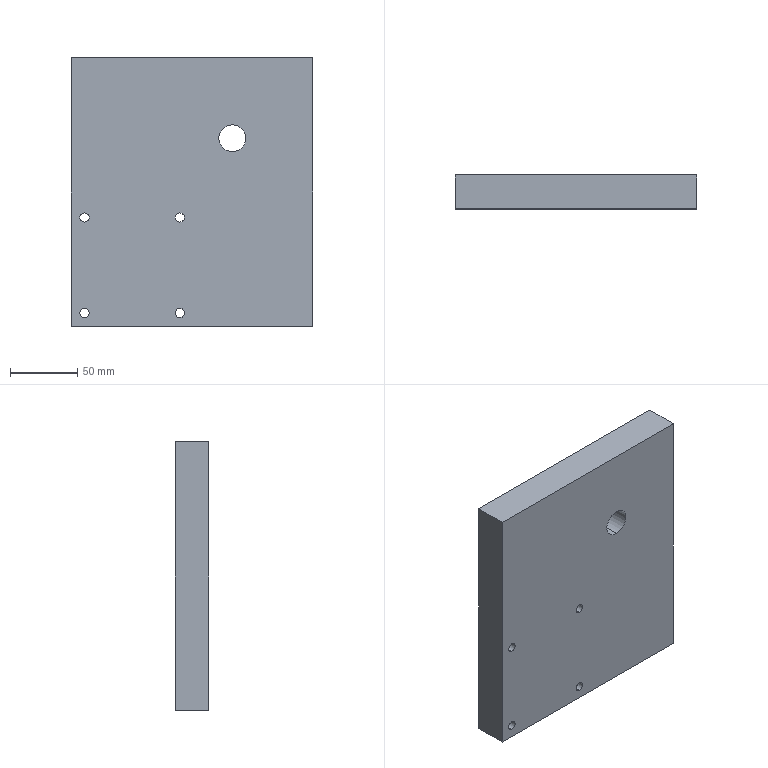Component | SolidWorks | 30-01A-1_Wheel-322-1_WheelFixingPlate-322-1 | 1 solid | 16 faces | box 180 x 25 x 200 mm | volume 888514 mm3 | cylinder 10 | plane 6 | commonest cylinder face diameters 6.8 x8 20 x2
build123d program:
from build123d import *

# Parameters (mm, degrees)
SKETCH1_W              = 200
SKETCH1_H              = 180
EXTRUDE1_DEPTH         = 12.5
M20X2_5_TAPPED_HOLE1_D = 20
M8X1_25_TAPPED_HOLE1_D = 6.8


with BuildPart() as part:
    # Sketch1 → Extrude1 (new, symmetric)
    with BuildSketch(Plane.XY):
        Rectangle(SKETCH1_W, SKETCH1_H)
    extrude(amount=EXTRUDE1_DEPTH, both=True)

    # M20x2.5 Tapped Hole1 (through all)
    with Locations(Plane.XY.offset(12.5)):
        with Locations((-40, -30)):
            Hole(M20X2_5_TAPPED_HOLE1_D / 2)

    # M8x1.25 Tapped Hole1 (through all)
    with Locations(Plane.XY.offset(12.5)):
        with Locations((19, 9), (90, 9), (90, 80), (19, 80)):
            Hole(M8X1_25_TAPPED_HOLE1_D / 2)


solid = part.part

# Placed as in the assembly
solid = solid.moved(Location((202.57, -550.345, -60), (-90, 0, 90)))
STEP:
#1=CARTESIAN_POINT('',(7.621,-22.159,-2.976));
#2=VERTEX_POINT('',#1);
#3=CARTESIAN_POINT('',(7.621,-22.159,-3.244));
#4=VERTEX_POINT('',#3);
#5=CARTESIAN_POINT('',(7.621,-22.159,-3.11));
#6=DIRECTION('',(0.,1.,-0.));
#7=DIRECTION('',(0.,0.,-1.));
#8=AXIS2_PLACEMENT_3D('',#5,#6,#7);
#9=CIRCLE('',#8,0.1339);
#10=EDGE_CURVE('',#2,#4,#9,.T.);
#11=ORIENTED_EDGE('',*,*,#10,.F.);
#12=CARTESIAN_POINT('',(7.621,-21.175,-2.976));
#13=VERTEX_POINT('',#12);
#14=CARTESIAN_POINT('',(7.621,-21.175,-2.976));
#15=DIRECTION('',(0.,1.,-0.));
#16=VECTOR('',#15,39.37);
#17=LINE('',#14,#16);
#18=EDGE_CURVE('',#2,#13,#17,.T.);
#19=ORIENTED_EDGE('',*,*,#18,.T.);
#20=CARTESIAN_POINT('',(7.621,-21.175,-3.244));
#21=VERTEX_POINT('',#20);
#22=CARTESIAN_POINT('',(7.621,-21.175,-3.11));
#23=DIRECTION('',(0.,1.,-0.));
#24=DIRECTION('',(0.,0.,-1.));
#25=AXIS2_PLACEMENT_3D('',#22,#23,#24);
#26=CIRCLE('',#25,0.1339);
#27=EDGE_CURVE('',#13,#21,#26,.T.);
#28=ORIENTED_EDGE('',*,*,#27,.T.);
#29=CARTESIAN_POINT('',(7.621,-21.175,-3.244));
#30=DIRECTION('',(0.,1.,-0.));
#31=VECTOR('',#30,39.37);
#32=LINE('',#29,#31);
#33=EDGE_CURVE('',#4,#21,#32,.T.);
#34=ORIENTED_EDGE('',*,*,#33,.F.);
#35=EDGE_LOOP('',(#11,#19,#28,#34));
#36=FACE_OUTER_BOUND('',#35,.T.);
#37=CARTESIAN_POINT('',(7.621,-21.175,-3.11));
#38=DIRECTION('',(0.,1.,-0.));
#39=DIRECTION('',(0.,0.,-1.));
#40=AXIS2_PLACEMENT_3D('',#37,#38,#39);
#41=CYLINDRICAL_SURFACE('',#40,0.1339);
#42=ADVANCED_FACE('',(#36),#41,.F.);
#43=CARTESIAN_POINT('',(7.621,-22.159,-5.772));
#44=VERTEX_POINT('',#43);
#45=CARTESIAN_POINT('',(7.621,-22.159,-6.039));
#46=VERTEX_POINT('',#45);
#47=CARTESIAN_POINT('',(7.621,-22.159,-5.906));
#48=DIRECTION('',(0.,1.,-0.));
#49=DIRECTION('',(0.,0.,-1.));
#50=AXIS2_PLACEMENT_3D('',#47,#48,#49);
#51=CIRCLE('',#50,0.1339);
#52=EDGE_CURVE('',#44,#46,#51,.T.);
#53=ORIENTED_EDGE('',*,*,#52,.F.);
#54=CARTESIAN_POINT('',(7.621,-21.175,-5.772));
#55=VERTEX_POINT('',#54);
#56=CARTESIAN_POINT('',(7.621,-21.175,-5.772));
#57=DIRECTION('',(0.,1.,-0.));
#58=VECTOR('',#57,39.37);
#59=LINE('',#56,#58);
#60=EDGE_CURVE('',#44,#55,#59,.T.);
#61=ORIENTED_EDGE('',*,*,#60,.T.);
#62=CARTESIAN_POINT('',(7.621,-21.175,-6.039));
#63=VERTEX_POINT('',#62);
#64=CARTESIAN_POINT('',(7.621,-21.175,-5.906));
#65=DIRECTION('',(0.,1.,-0.));
#66=DIRECTION('',(0.,0.,-1.));
#67=AXIS2_PLACEMENT_3D('',#64,#65,#66);
#68=CIRCLE('',#67,0.1339);
#69=EDGE_CURVE('',#55,#63,#68,.T.);
#70=ORIENTED_EDGE('',*,*,#69,.T.);
#71=CARTESIAN_POINT('',(7.621,-21.175,-6.039));
#72=DIRECTION('',(0.,1.,-0.));
#73=VECTOR('',#72,39.37);
#74=LINE('',#71,#73);
#75=EDGE_CURVE('',#46,#63,#74,.T.);
#76=ORIENTED_EDGE('',*,*,#75,.F.);
#77=EDGE_LOOP('',(#53,#61,#70,#76));
#78=FACE_OUTER_BOUND('',#77,.T.);
#79=CARTESIAN_POINT('',(7.621,-21.175,-5.906));
#80=DIRECTION('',(0.,1.,-0.));
#81=DIRECTION('',(0.,0.,-1.));
#82=AXIS2_PLACEMENT_3D('',#79,#80,#81);
#83=CYLINDRICAL_SURFACE('',#82,0.1339);
#84=ADVANCED_FACE('',(#78),#83,.F.);
#85=CARTESIAN_POINT('',(4.826,-22.159,-5.772));
#86=VERTEX_POINT('',#85);
#87=CARTESIAN_POINT('',(4.826,-22.159,-6.039));
#88=VERTEX_POINT('',#87);
#89=CARTESIAN_POINT('',(4.826,-22.159,-5.906));
#90=DIRECTION('',(0.,1.,-0.));
#91=DIRECTION('',(0.,0.,-1.));
#92=AXIS2_PLACEMENT_3D('',#89,#90,#91);
#93=CIRCLE('',#92,0.1339);
#94=EDGE_CURVE('',#86,#88,#93,.T.);
#95=ORIENTED_EDGE('',*,*,#94,.F.);
#96=CARTESIAN_POINT('',(4.826,-21.175,-5.772));
#97=VERTEX_POINT('',#96);
#98=CARTESIAN_POINT('',(4.826,-21.175,-5.772));
#99=DIRECTION('',(0.,1.,-0.));
#100=VECTOR('',#99,39.37);
#101=LINE('',#98,#100);
#102=EDGE_CURVE('',#86,#97,#101,.T.);
#103=ORIENTED_EDGE('',*,*,#102,.T.);
#104=CARTESIAN_POINT('',(4.826,-21.175,-6.039));
#105=VERTEX_POINT('',#104);
#106=CARTESIAN_POINT('',(4.826,-21.175,-5.906));
#107=DIRECTION('',(0.,1.,-0.));
#108=DIRECTION('',(0.,0.,-1.));
#109=AXIS2_PLACEMENT_3D('',#106,#107,#108);
#110=CIRCLE('',#109,0.1339);
#111=EDGE_CURVE('',#97,#105,#110,.T.);
#112=ORIENTED_EDGE('',*,*,#111,.T.);
#113=CARTESIAN_POINT('',(4.826,-21.175,-6.039));
#114=DIRECTION('',(0.,1.,-0.));
#115=VECTOR('',#114,39.37);
#116=LINE('',#113,#115);
#117=EDGE_CURVE('',#88,#105,#116,.T.);
#118=ORIENTED_EDGE('',*,*,#117,.F.);
#119=EDGE_LOOP('',(#95,#103,#112,#118));
#120=FACE_OUTER_BOUND('',#119,.T.);
#121=CARTESIAN_POINT('',(4.826,-21.175,-5.906));
#122=DIRECTION('',(0.,1.,-0.));
#123=DIRECTION('',(0.,0.,-1.));
#124=AXIS2_PLACEMENT_3D('',#121,#122,#123);
#125=CYLINDRICAL_SURFACE('',#124,0.1339);
#126=ADVANCED_FACE('',(#120),#125,.F.);
#127=CARTESIAN_POINT('',(4.826,-22.159,-2.976));
#128=VERTEX_POINT('',#127);
#129=CARTESIAN_POINT('',(4.826,-22.159,-3.244));
#130=VERTEX_POINT('',#129);
#131=CARTESIAN_POINT('',(4.826,-22.159,-3.11));
#132=DIRECTION('',(0.,1.,-0.));
#133=DIRECTION('',(0.,0.,-1.));
#134=AXIS2_PLACEMENT_3D('',#131,#132,#133);
#135=CIRCLE('',#134,0.1339);
#136=EDGE_CURVE('',#128,#130,#135,.T.);
#137=ORIENTED_EDGE('',*,*,#136,.F.);
#138=CARTESIAN_POINT('',(4.826,-21.175,-2.976));
#139=VERTEX_POINT('',#138);
#140=CARTESIAN_POINT('',(4.826,-21.175,-2.976));
#141=DIRECTION('',(0.,1.,-0.));
#142=VECTOR('',#141,39.37);
#143=LINE('',#140,#142);
#144=EDGE_CURVE('',#128,#139,#143,.T.);
#145=ORIENTED_EDGE('',*,*,#144,.T.);
#146=CARTESIAN_POINT('',(4.826,-21.175,-3.244));
#147=VERTEX_POINT('',#146);
#148=CARTESIAN_POINT('',(4.826,-21.175,-3.11));
#149=DIRECTION('',(0.,1.,-0.));
#150=DIRECTION('',(0.,0.,-1.));
#151=AXIS2_PLACEMENT_3D('',#148,#149,#150);
#152=CIRCLE('',#151,0.1339);
#153=EDGE_CURVE('',#139,#147,#152,.T.);
#154=ORIENTED_EDGE('',*,*,#153,.T.);
#155=CARTESIAN_POINT('',(4.826,-21.175,-3.244));
#156=DIRECTION('',(0.,1.,-0.));
#157=VECTOR('',#156,39.37);
#158=LINE('',#155,#157);
#159=EDGE_CURVE('',#130,#147,#158,.T.);
#160=ORIENTED_EDGE('',*,*,#159,.F.);
#161=EDGE_LOOP('',(#137,#145,#154,#160));
#162=FACE_OUTER_BOUND('',#161,.T.);
#163=CARTESIAN_POINT('',(4.826,-21.175,-3.11));
#164=DIRECTION('',(0.,1.,-0.));
#165=DIRECTION('',(0.,0.,-1.));
#166=AXIS2_PLACEMENT_3D('',#163,#164,#165);
#167=CYLINDRICAL_SURFACE('',#166,0.1339);
#168=ADVANCED_FACE('',(#162),#167,.F.);
#169=CARTESIAN_POINT('',(9.156,-22.159,-0.3937));
#170=VERTEX_POINT('',#169);
#171=CARTESIAN_POINT('',(9.156,-22.159,-1.181));
#172=VERTEX_POINT('',#171);
#173=CARTESIAN_POINT('',(9.156,-22.159,-0.7874));
#174=DIRECTION('',(0.,1.,-0.));
#175=DIRECTION('',(0.,0.,-1.));
#176=AXIS2_PLACEMENT_3D('',#173,#174,#175);
#177=CIRCLE('',#176,0.3937);
#178=EDGE_CURVE('',#170,#172,#177,.T.);
#179=ORIENTED_EDGE('',*,*,#178,.F.);
#180=CARTESIAN_POINT('',(9.156,-21.175,-0.3937));
#181=VERTEX_POINT('',#180);
#182=CARTESIAN_POINT('',(9.156,-21.175,-0.3937));
#183=DIRECTION('',(0.,1.,-0.));
#184=VECTOR('',#183,39.37);
#185=LINE('',#182,#184);
#186=EDGE_CURVE('',#170,#181,#185,.T.);
#187=ORIENTED_EDGE('',*,*,#186,.T.);
#188=CARTESIAN_POINT('',(9.156,-21.175,-1.181));
#189=VERTEX_POINT('',#188);
#190=CARTESIAN_POINT('',(9.156,-21.175,-0.7874));
#191=DIRECTION('',(0.,1.,-0.));
#192=DIRECTION('',(0.,0.,-1.));
#193=AXIS2_PLACEMENT_3D('',#190,#191,#192);
#194=CIRCLE('',#193,0.3937);
#195=EDGE_CURVE('',#181,#189,#194,.T.);
#196=ORIENTED_EDGE('',*,*,#195,.T.);
#197=CARTESIAN_POINT('',(9.156,-21.175,-1.181));
#198=DIRECTION('',(0.,1.,-0.));
#199=VECTOR('',#198,39.37);
#200=LINE('',#197,#199);
#201=EDGE_CURVE('',#172,#189,#200,.T.);
#202=ORIENTED_EDGE('',*,*,#201,.F.);
#203=EDGE_LOOP('',(#179,#187,#196,#202));
#204=FACE_OUTER_BOUND('',#203,.T.);
#205=CARTESIAN_POINT('',(9.156,-21.175,-0.7874));
#206=DIRECTION('',(0.,1.,-0.));
#207=DIRECTION('',(0.,0.,-1.));
#208=AXIS2_PLACEMENT_3D('',#205,#206,#207);
#209=CYLINDRICAL_SURFACE('',#208,0.3937);
#210=ADVANCED_FACE('',(#204),#209,.F.);
#211=CARTESIAN_POINT('',(4.432,-22.159,1.575));
#212=VERTEX_POINT('',#211);
#213=CARTESIAN_POINT('',(11.519,-22.159,1.575));
#214=VERTEX_POINT('',#213);
#215=CARTESIAN_POINT('',(4.432,-22.159,1.575));
#216=DIRECTION('',(1.,-0.,-0.));
#217=VECTOR('',#216,39.37);
#218=LINE('',#215,#217);
#219=EDGE_CURVE('',#212,#214,#218,.T.);
#220=ORIENTED_EDGE('',*,*,#219,.T.);
#221=CARTESIAN_POINT('',(11.519,-21.175,1.575));
#222=VERTEX_POINT('',#221);
#223=CARTESIAN_POINT('',(11.519,-21.175,1.575));
#224=DIRECTION('',(-0.,-1.,0.));
#225=VECTOR('',#224,39.37);
#226=LINE('',#223,#225);
#227=EDGE_CURVE('',#222,#214,#226,.T.);
#228=ORIENTED_EDGE('',*,*,#227,.F.);
#229=CARTESIAN_POINT('',(4.432,-21.175,1.575));
#230=VERTEX_POINT('',#229);
#231=CARTESIAN_POINT('',(4.432,-21.175,1.575));
#232=DIRECTION('',(1.,-0.,-0.));
#233=VECTOR('',#232,39.37);
#234=LINE('',#231,#233);
#235=EDGE_CURVE('',#230,#222,#234,.T.);
#236=ORIENTED_EDGE('',*,*,#235,.F.);
#237=CARTESIAN_POINT('',(4.432,-21.175,1.575));
#238=DIRECTION('',(-0.,-1.,0.));
#239=VECTOR('',#238,39.37);
#240=LINE('',#237,#239);
#241=EDGE_CURVE('',#230,#212,#240,.T.);
#242=ORIENTED_EDGE('',*,*,#241,.T.);
#243=EDGE_LOOP('',(#220,#228,#236,#242));
#244=FACE_OUTER_BOUND('',#243,.T.);
#245=CARTESIAN_POINT('',(4.432,-21.175,1.575));
#246=DIRECTION('',(-0.,-0.,-1.));
#247=DIRECTION('',(-0.,-1.,0.));
#248=AXIS2_PLACEMENT_3D('',#245,#246,#247);
#249=PLANE('',#248);
#250=ADVANCED_FACE('',(#244),#249,.F.);
#251=CARTESIAN_POINT('',(11.519,-22.159,-6.299));
#252=VERTEX_POINT('',#251);
#253=CARTESIAN_POINT('',(11.519,-22.159,1.575));
#254=DIRECTION('',(-0.,-0.,-1.));
#255=VECTOR('',#254,39.37);
#256=LINE('',#253,#255);
#257=EDGE_CURVE('',#214,#252,#256,.T.);
#258=ORIENTED_EDGE('',*,*,#257,.T.);
#259=CARTESIAN_POINT('',(11.519,-21.175,-6.299));
#260=VERTEX_POINT('',#259);
#261=CARTESIAN_POINT('',(11.519,-21.175,-6.299));
#262=DIRECTION('',(-0.,-1.,0.));
#263=VECTOR('',#262,39.37);
#264=LINE('',#261,#263);
#265=EDGE_CURVE('',#260,#252,#264,.T.);
#266=ORIENTED_EDGE('',*,*,#265,.F.);
#267=CARTESIAN_POINT('',(11.519,-21.175,1.575));
#268=DIRECTION('',(-0.,-0.,-1.));
#269=VECTOR('',#268,39.37);
#270=LINE('',#267,#269);
#271=EDGE_CURVE('',#222,#260,#270,.T.);
#272=ORIENTED_EDGE('',*,*,#271,.F.);
#273=ORIENTED_EDGE('',*,*,#227,.T.);
#274=EDGE_LOOP('',(#258,#266,#272,#273));
#275=FACE_OUTER_BOUND('',#274,.T.);
#276=CARTESIAN_POINT('',(11.519,-21.175,1.575));
#277=DIRECTION('',(-1.,0.,0.));
#278=DIRECTION('',(0.,1.,-0.));
#279=AXIS2_PLACEMENT_3D('',#276,#277,#278);
#280=PLANE('',#279);
#281=ADVANCED_FACE('',(#275),#280,.F.);
#282=CARTESIAN_POINT('',(4.432,-22.159,-6.299));
#283=VERTEX_POINT('',#282);
#284=CARTESIAN_POINT('',(4.432,-22.159,-6.299));
#285=DIRECTION('',(-1.,0.,0.));
#286=VECTOR('',#285,39.37);
#287=LINE('',#284,#286);
#288=EDGE_CURVE('',#252,#283,#287,.T.);
#289=ORIENTED_EDGE('',*,*,#288,.T.);
#290=CARTESIAN_POINT('',(4.432,-21.175,-6.299));
#291=VERTEX_POINT('',#290);
#292=CARTESIAN_POINT('',(4.432,-21.175,-6.299));
#293=DIRECTION('',(-0.,-1.,0.));
#294=VECTOR('',#293,39.37);
#295=LINE('',#292,#294);
#296=EDGE_CURVE('',#291,#283,#295,.T.);
#297=ORIENTED_EDGE('',*,*,#296,.F.);
#298=CARTESIAN_POINT('',(4.432,-21.175,-6.299));
#299=DIRECTION('',(-1.,0.,0.));
#300=VECTOR('',#299,39.37);
#301=LINE('',#298,#300);
#302=EDGE_CURVE('',#260,#291,#301,.T.);
#303=ORIENTED_EDGE('',*,*,#302,.F.);
#304=ORIENTED_EDGE('',*,*,#265,.T.);
#305=EDGE_LOOP('',(#289,#297,#303,#304));
#306=FACE_OUTER_BOUND('',#305,.T.);
#307=CARTESIAN_POINT('',(4.432,-21.175,-6.299));
#308=DIRECTION('',(0.,0.,1.));
#309=DIRECTION('',(0.,1.,-0.));
#310=AXIS2_PLACEMENT_3D('',#307,#308,#309);
#311=PLANE('',#310);
#312=ADVANCED_FACE('',(#306),#311,.F.);
#313=CARTESIAN_POINT('',(4.432,-22.159,1.575));
#314=DIRECTION('',(0.,0.,1.));
#315=VECTOR('',#314,39.37);
#316=LINE('',#313,#315);
#317=EDGE_CURVE('',#283,#212,#316,.T.);
#318=ORIENTED_EDGE('',*,*,#317,.T.);
#319=ORIENTED_EDGE('',*,*,#241,.F.);
#320=CARTESIAN_POINT('',(4.432,-21.175,1.575));
#321=DIRECTION('',(0.,0.,1.));
#322=VECTOR('',#321,39.37);
#323=LINE('',#320,#322);
#324=EDGE_CURVE('',#291,#230,#323,.T.);
#325=ORIENTED_EDGE('',*,*,#324,.F.);
#326=ORIENTED_EDGE('',*,*,#296,.T.);
#327=EDGE_LOOP('',(#318,#319,#325,#326));
#328=FACE_OUTER_BOUND('',#327,.T.);
#329=CARTESIAN_POINT('',(4.432,-21.175,1.575));
#330=DIRECTION('',(1.,-0.,-0.));
#331=DIRECTION('',(-0.,-1.,0.));
#332=AXIS2_PLACEMENT_3D('',#329,#330,#331);
#333=PLANE('',#332);
#334=ADVANCED_FACE('',(#328),#333,.F.);
#335=CARTESIAN_POINT('',(7.621,-21.175,-3.11));
#336=DIRECTION('',(0.,1.,-0.));
#337=DIRECTION('',(0.,0.,-1.));
#338=AXIS2_PLACEMENT_3D('',#335,#336,#337);
#339=CIRCLE('',#338,0.1339);
#340=EDGE_CURVE('',#21,#13,#339,.T.);
#341=ORIENTED_EDGE('',*,*,#340,.F.);
#342=ORIENTED_EDGE('',*,*,#27,.F.);
#343=EDGE_LOOP('',(#341,#342));
#344=FACE_BOUND('',#343,.T.);
#345=CARTESIAN_POINT('',(7.621,-21.175,-5.906));
#346=DIRECTION('',(0.,1.,-0.));
#347=DIRECTION('',(0.,0.,-1.));
#348=AXIS2_PLACEMENT_3D('',#345,#346,#347);
#349=CIRCLE('',#348,0.1339);
#350=EDGE_CURVE('',#63,#55,#349,.T.);
#351=ORIENTED_EDGE('',*,*,#350,.F.);
#352=ORIENTED_EDGE('',*,*,#69,.F.);
#353=EDGE_LOOP('',(#351,#352));
#354=FACE_BOUND('',#353,.T.);
#355=CARTESIAN_POINT('',(4.826,-21.175,-5.906));
#356=DIRECTION('',(0.,1.,-0.));
#357=DIRECTION('',(0.,0.,-1.));
#358=AXIS2_PLACEMENT_3D('',#355,#356,#357);
#359=CIRCLE('',#358,0.1339);
#360=EDGE_CURVE('',#105,#97,#359,.T.);
#361=ORIENTED_EDGE('',*,*,#360,.F.);
#362=ORIENTED_EDGE('',*,*,#111,.F.);
#363=EDGE_LOOP('',(#361,#362));
#364=FACE_BOUND('',#363,.T.);
#365=CARTESIAN_POINT('',(4.826,-21.175,-3.11));
#366=DIRECTION('',(0.,1.,-0.));
#367=DIRECTION('',(0.,0.,-1.));
#368=AXIS2_PLACEMENT_3D('',#365,#366,#367);
#369=CIRCLE('',#368,0.1339);
#370=EDGE_CURVE('',#147,#139,#369,.T.);
#371=ORIENTED_EDGE('',*,*,#370,.F.);
#372=ORIENTED_EDGE('',*,*,#153,.F.);
#373=EDGE_LOOP('',(#371,#372));
#374=FACE_BOUND('',#373,.T.);
#375=CARTESIAN_POINT('',(9.156,-21.175,-0.7874));
#376=DIRECTION('',(0.,1.,-0.));
#377=DIRECTION('',(0.,0.,-1.));
#378=AXIS2_PLACEMENT_3D('',#375,#376,#377);
#379=CIRCLE('',#378,0.3937);
#380=EDGE_CURVE('',#189,#181,#379,.T.);
#381=ORIENTED_EDGE('',*,*,#380,.F.);
#382=ORIENTED_EDGE('',*,*,#195,.F.);
#383=EDGE_LOOP('',(#381,#382));
#384=FACE_BOUND('',#383,.T.);
#385=ORIENTED_EDGE('',*,*,#235,.T.);
#386=ORIENTED_EDGE('',*,*,#271,.T.);
#387=ORIENTED_EDGE('',*,*,#302,.T.);
#388=ORIENTED_EDGE('',*,*,#324,.T.);
#389=EDGE_LOOP('',(#385,#386,#387,#388));
#390=FACE_OUTER_BOUND('',#389,.T.);
#391=CARTESIAN_POINT('',(11.519,-21.175,1.575));
#392=DIRECTION('',(0.,1.,-0.));
#393=DIRECTION('',(-0.,-0.,-1.));
#394=AXIS2_PLACEMENT_3D('',#391,#392,#393);
#395=PLANE('',#394);
#396=ADVANCED_FACE('',(#344,#354,#364,#374,#384,#390),#395,.T.);
#397=CARTESIAN_POINT('',(7.621,-22.159,-3.11));
#398=DIRECTION('',(0.,1.,-0.));
#399=DIRECTION('',(0.,0.,-1.));
#400=AXIS2_PLACEMENT_3D('',#397,#398,#399);
#401=CIRCLE('',#400,0.1339);
#402=EDGE_CURVE('',#4,#2,#401,.T.);
#403=ORIENTED_EDGE('',*,*,#402,.T.);
#404=ORIENTED_EDGE('',*,*,#10,.T.);
#405=EDGE_LOOP('',(#403,#404));
#406=FACE_BOUND('',#405,.T.);
#407=CARTESIAN_POINT('',(7.621,-22.159,-5.906));
#408=DIRECTION('',(0.,1.,-0.));
#409=DIRECTION('',(0.,0.,-1.));
#410=AXIS2_PLACEMENT_3D('',#407,#408,#409);
#411=CIRCLE('',#410,0.1339);
#412=EDGE_CURVE('',#46,#44,#411,.T.);
#413=ORIENTED_EDGE('',*,*,#412,.T.);
#414=ORIENTED_EDGE('',*,*,#52,.T.);
#415=EDGE_LOOP('',(#413,#414));
#416=FACE_BOUND('',#415,.T.);
#417=CARTESIAN_POINT('',(4.826,-22.159,-5.906));
#418=DIRECTION('',(0.,1.,-0.));
#419=DIRECTION('',(0.,0.,-1.));
#420=AXIS2_PLACEMENT_3D('',#417,#418,#419);
#421=CIRCLE('',#420,0.1339);
#422=EDGE_CURVE('',#88,#86,#421,.T.);
#423=ORIENTED_EDGE('',*,*,#422,.T.);
#424=ORIENTED_EDGE('',*,*,#94,.T.);
#425=EDGE_LOOP('',(#423,#424));
#426=FACE_BOUND('',#425,.T.);
#427=CARTESIAN_POINT('',(4.826,-22.159,-3.11));
#428=DIRECTION('',(0.,1.,-0.));
#429=DIRECTION('',(0.,0.,-1.));
#430=AXIS2_PLACEMENT_3D('',#427,#428,#429);
#431=CIRCLE('',#430,0.1339);
#432=EDGE_CURVE('',#130,#128,#431,.T.);
#433=ORIENTED_EDGE('',*,*,#432,.T.);
#434=ORIENTED_EDGE('',*,*,#136,.T.);
#435=EDGE_LOOP('',(#433,#434));
#436=FACE_BOUND('',#435,.T.);
#437=CARTESIAN_POINT('',(9.156,-22.159,-0.7874));
#438=DIRECTION('',(0.,1.,-0.));
#439=DIRECTION('',(0.,0.,-1.));
#440=AXIS2_PLACEMENT_3D('',#437,#438,#439);
#441=CIRCLE('',#440,0.3937);
#442=EDGE_CURVE('',#172,#170,#441,.T.);
#443=ORIENTED_EDGE('',*,*,#442,.T.);
#444=ORIENTED_EDGE('',*,*,#178,.T.);
#445=EDGE_LOOP('',(#443,#444));
#446=FACE_BOUND('',#445,.T.);
#447=ORIENTED_EDGE('',*,*,#219,.F.);
#448=ORIENTED_EDGE('',*,*,#317,.F.);
#449=ORIENTED_EDGE('',*,*,#288,.F.);
#450=ORIENTED_EDGE('',*,*,#257,.F.);
#451=EDGE_LOOP('',(#447,#448,#449,#450));
#452=FACE_OUTER_BOUND('',#451,.T.);
#453=CARTESIAN_POINT('',(11.519,-22.159,1.575));
#454=DIRECTION('',(0.,1.,-0.));
#455=DIRECTION('',(-0.,-0.,-1.));
#456=AXIS2_PLACEMENT_3D('',#453,#454,#455);
#457=PLANE('',#456);
#458=ADVANCED_FACE('',(#406,#416,#426,#436,#446,#452),#457,.F.);
#459=ORIENTED_EDGE('',*,*,#186,.F.);
#460=ORIENTED_EDGE('',*,*,#442,.F.);
#461=ORIENTED_EDGE('',*,*,#201,.T.);
#462=ORIENTED_EDGE('',*,*,#380,.T.);
#463=EDGE_LOOP('',(#459,#460,#461,#462));
#464=FACE_OUTER_BOUND('',#463,.T.);
#465=CARTESIAN_POINT('',(9.156,-21.175,-0.7874));
#466=DIRECTION('',(0.,1.,-0.));
#467=DIRECTION('',(0.,0.,-1.));
#468=AXIS2_PLACEMENT_3D('',#465,#466,#467);
#469=CYLINDRICAL_SURFACE('',#468,0.3937);
#470=ADVANCED_FACE('',(#464),#469,.F.);
#471=ORIENTED_EDGE('',*,*,#144,.F.);
#472=ORIENTED_EDGE('',*,*,#432,.F.);
#473=ORIENTED_EDGE('',*,*,#159,.T.);
#474=ORIENTED_EDGE('',*,*,#370,.T.);
#475=EDGE_LOOP('',(#471,#472,#473,#474));
#476=FACE_OUTER_BOUND('',#475,.T.);
#477=CARTESIAN_POINT('',(4.826,-21.175,-3.11));
#478=DIRECTION('',(0.,1.,-0.));
#479=DIRECTION('',(0.,0.,-1.));
#480=AXIS2_PLACEMENT_3D('',#477,#478,#479);
#481=CYLINDRICAL_SURFACE('',#480,0.1339);
#482=ADVANCED_FACE('',(#476),#481,.F.);
#483=ORIENTED_EDGE('',*,*,#102,.F.);
#484=ORIENTED_EDGE('',*,*,#422,.F.);
#485=ORIENTED_EDGE('',*,*,#117,.T.);
#486=ORIENTED_EDGE('',*,*,#360,.T.);
#487=EDGE_LOOP('',(#483,#484,#485,#486));
#488=FACE_OUTER_BOUND('',#487,.T.);
#489=CARTESIAN_POINT('',(4.826,-21.175,-5.906));
#490=DIRECTION('',(0.,1.,-0.));
#491=DIRECTION('',(0.,0.,-1.));
#492=AXIS2_PLACEMENT_3D('',#489,#490,#491);
#493=CYLINDRICAL_SURFACE('',#492,0.1339);
#494=ADVANCED_FACE('',(#488),#493,.F.);
#495=ORIENTED_EDGE('',*,*,#60,.F.);
#496=ORIENTED_EDGE('',*,*,#412,.F.);
#497=ORIENTED_EDGE('',*,*,#75,.T.);
#498=ORIENTED_EDGE('',*,*,#350,.T.);
#499=EDGE_LOOP('',(#495,#496,#497,#498));
#500=FACE_OUTER_BOUND('',#499,.T.);
#501=CARTESIAN_POINT('',(7.621,-21.175,-5.906));
#502=DIRECTION('',(0.,1.,-0.));
#503=DIRECTION('',(0.,0.,-1.));
#504=AXIS2_PLACEMENT_3D('',#501,#502,#503);
#505=CYLINDRICAL_SURFACE('',#504,0.1339);
#506=ADVANCED_FACE('',(#500),#505,.F.);
#507=ORIENTED_EDGE('',*,*,#18,.F.);
#508=ORIENTED_EDGE('',*,*,#402,.F.);
#509=ORIENTED_EDGE('',*,*,#33,.T.);
#510=ORIENTED_EDGE('',*,*,#340,.T.);
#511=EDGE_LOOP('',(#507,#508,#509,#510));
#512=FACE_OUTER_BOUND('',#511,.T.);
#513=CARTESIAN_POINT('',(7.621,-21.175,-3.11));
#514=DIRECTION('',(0.,1.,-0.));
#515=DIRECTION('',(0.,0.,-1.));
#516=AXIS2_PLACEMENT_3D('',#513,#514,#515);
#517=CYLINDRICAL_SURFACE('',#516,0.1339);
#518=ADVANCED_FACE('',(#512),#517,.F.);
#519=CLOSED_SHELL('',(#42,#84,#126,#168,#210,#250,#281,#312,#334,#396,#458,#470,#482,#494,#506,#518));
#520=MANIFOLD_SOLID_BREP('',#519);
#521=CARTESIAN_POINT('',(0.,0.,0.));
#522=DIRECTION('',(0.,0.,1.));
#523=DIRECTION('',(1.,0.,0.));
#524=AXIS2_PLACEMENT_3D('',#521,#522,#523);
#525=(LENGTH_UNIT()NAMED_UNIT(*)SI_UNIT($,.METRE.));
#526=LENGTH_MEASURE_WITH_UNIT(LENGTH_MEASURE(0.0254),#525);
#527=DIMENSIONAL_EXPONENTS(1.,0.,0.,0.,0.,0.,0.);
#528=(CONVERSION_BASED_UNIT('',#526)LENGTH_UNIT()NAMED_UNIT(#527));
#529=UNCERTAINTY_MEASURE_WITH_UNIT(LENGTH_MEASURE(0.00001),#528,'','');
#530=(NAMED_UNIT(*)PLANE_ANGLE_UNIT()SI_UNIT($,.RADIAN.));
#531=(NAMED_UNIT(*)SI_UNIT($,.STERADIAN.)SOLID_ANGLE_UNIT());
#532=(GEOMETRIC_REPRESENTATION_CONTEXT(3)GLOBAL_UNCERTAINTY_ASSIGNED_CONTEXT((#529))GLOBAL_UNIT_ASSIGNED_CONTEXT((#528,#530,#531))REPRESENTATION_CONTEXT('',''));
#533=ADVANCED_BREP_SHAPE_REPRESENTATION('',(#520,#524),#532);
#534=COLOUR_RGB('',0.7922,0.8196,0.9333);
#535=FILL_AREA_STYLE_COLOUR('',#534);
#536=FILL_AREA_STYLE('',(#535));
#537=SURFACE_STYLE_FILL_AREA(#536);
#538=SURFACE_SIDE_STYLE('',(#537));
#539=SURFACE_STYLE_USAGE(.BOTH.,#538);
#540=PRESENTATION_STYLE_ASSIGNMENT((#539));
#541=STYLED_ITEM('',(#540),#520);
#542=PRESENTATION_LAYER_ASSIGNMENT('','',(#541));
#543=(LENGTH_UNIT()NAMED_UNIT(*)SI_UNIT($,.METRE.));
#544=LENGTH_MEASURE_WITH_UNIT(LENGTH_MEASURE(0.0254),#543);
#545=DIMENSIONAL_EXPONENTS(1.,0.,0.,0.,0.,0.,0.);
#546=(CONVERSION_BASED_UNIT('',#544)LENGTH_UNIT()NAMED_UNIT(#545));
#547=UNCERTAINTY_MEASURE_WITH_UNIT(LENGTH_MEASURE(0.00001),#546,'','');
#548=(NAMED_UNIT(*)PLANE_ANGLE_UNIT()SI_UNIT($,.RADIAN.));
#549=(NAMED_UNIT(*)SI_UNIT($,.STERADIAN.)SOLID_ANGLE_UNIT());
#550=(GEOMETRIC_REPRESENTATION_CONTEXT(3)GLOBAL_UNCERTAINTY_ASSIGNED_CONTEXT((#547))GLOBAL_UNIT_ASSIGNED_CONTEXT((#546,#548,#549))REPRESENTATION_CONTEXT('',''));
#551=MECHANICAL_DESIGN_GEOMETRIC_PRESENTATION_REPRESENTATION('',(#541),#550);